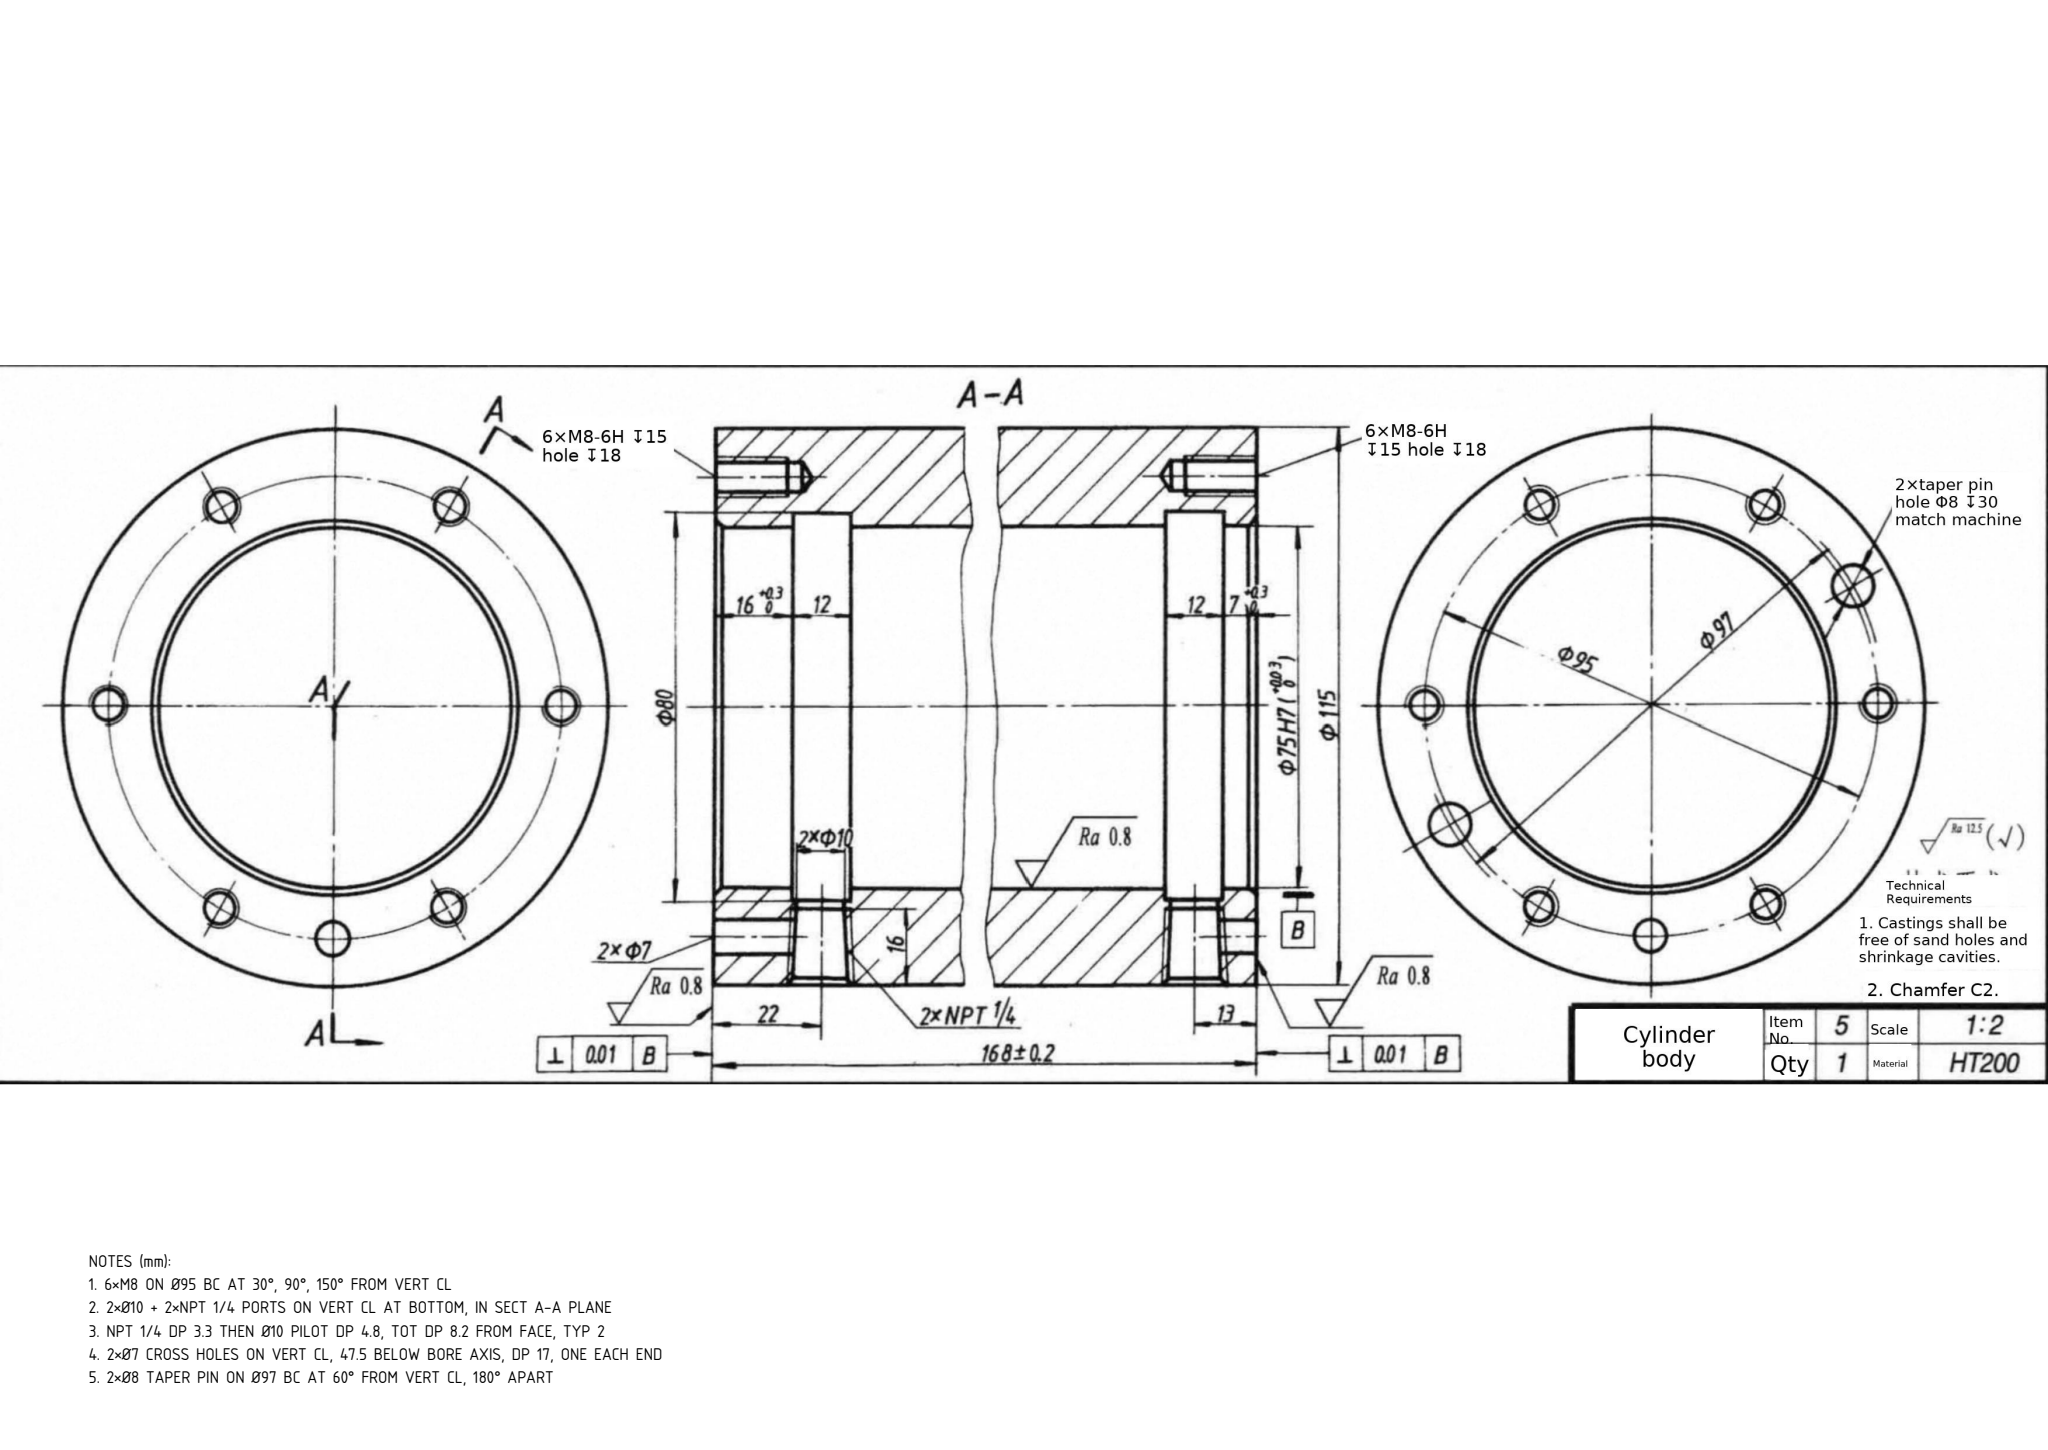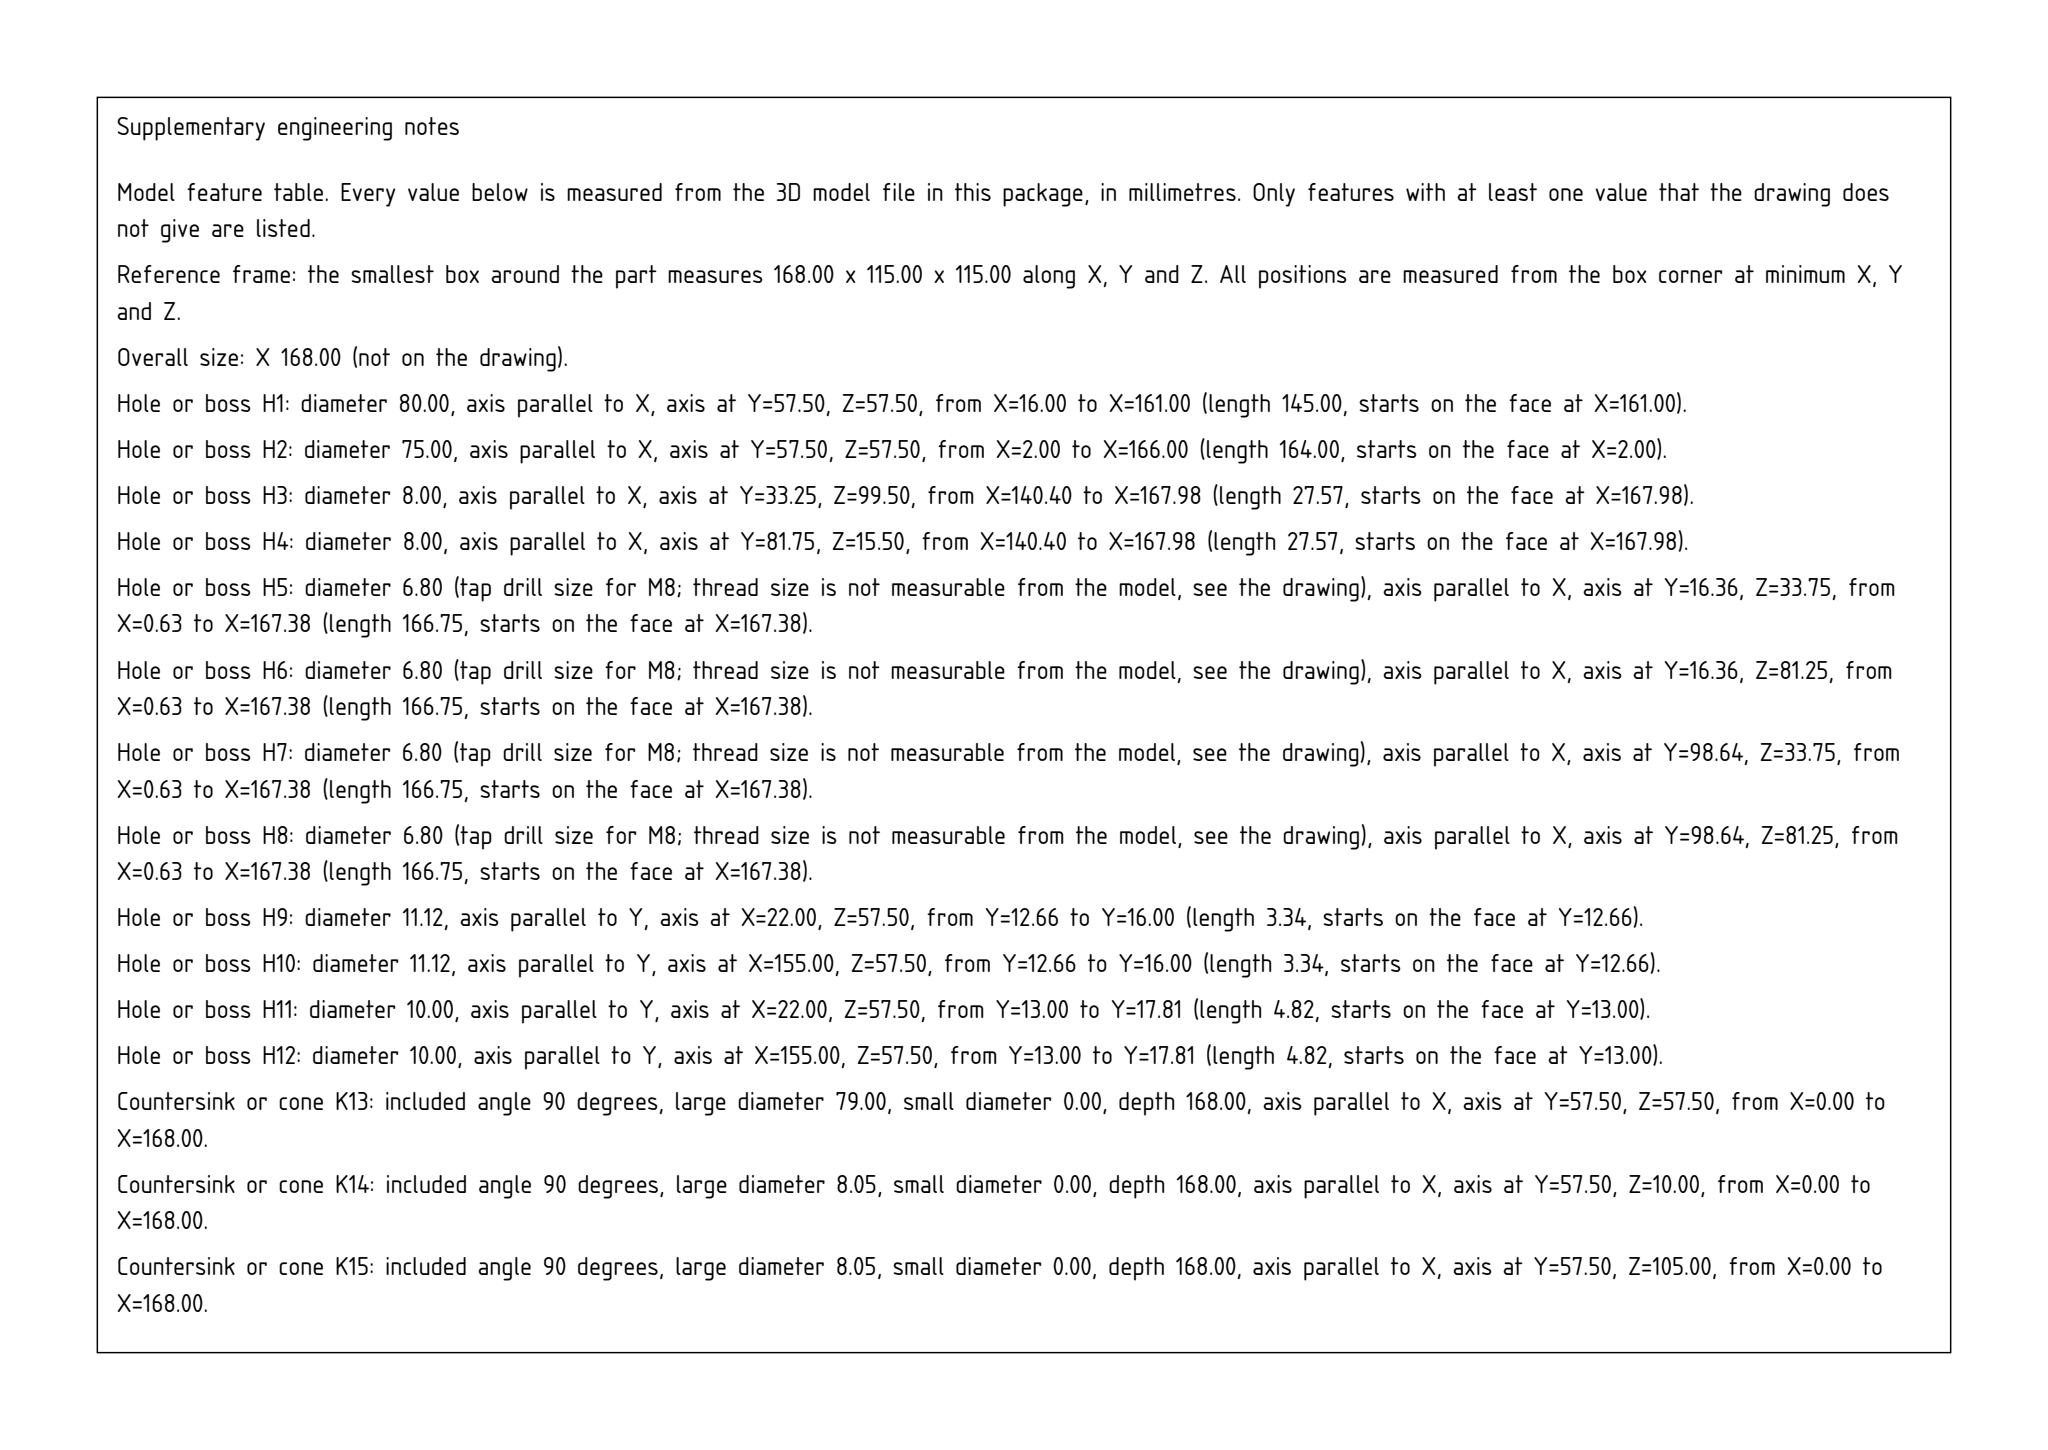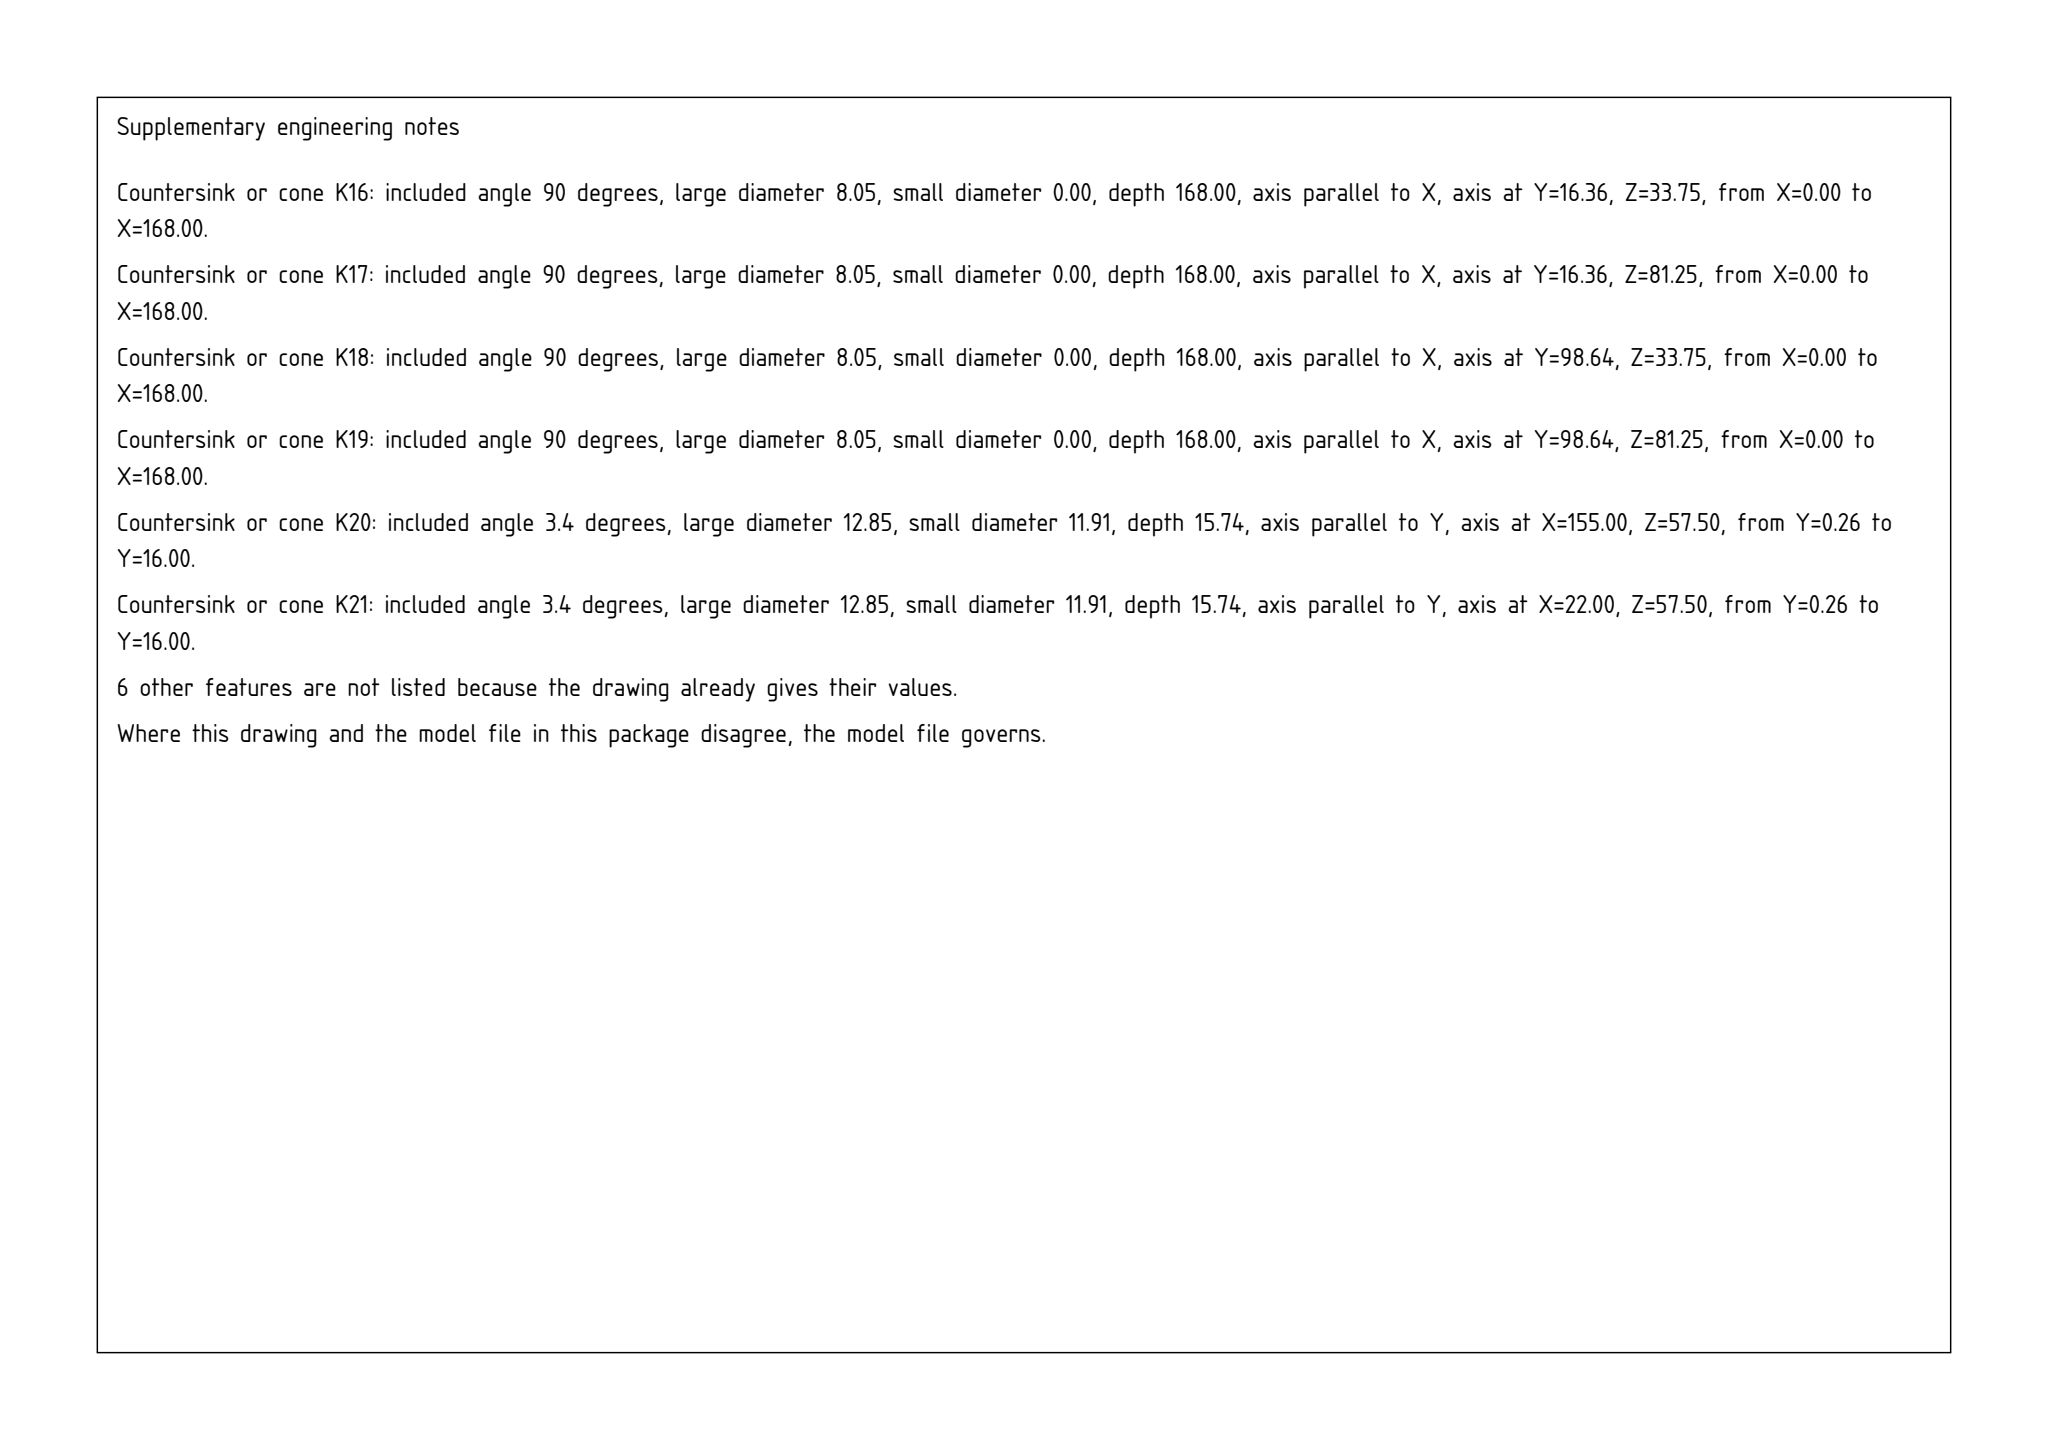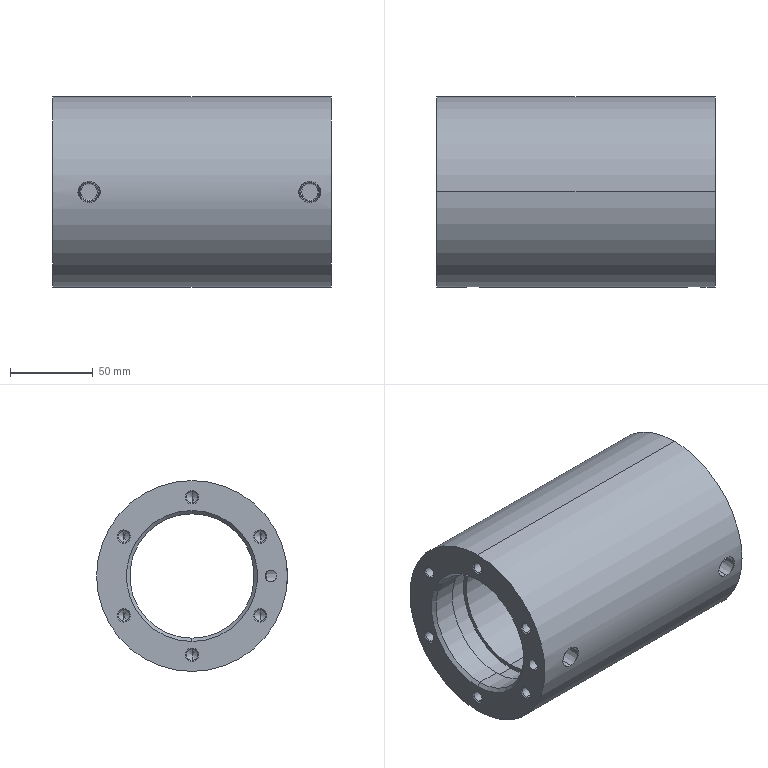Part | SolidWorks | mm | 1 solid | 136 faces | box 168 x 115 x 115 mm | volume 972210 mm3 | cone 74 | cylinder 54 | plane 8 | commonest cylinder face diameters 6.8 x24 7 x6 75 x6 10 x4 11.125 x4 8 x4 80 x4 115 x2
Drawing notes:
6×M8 ON Ø95 BC AT 30°, 90°, 150° FROM VERT CL | from the solid: 6×Ø6.8 tap drills at (16.36,33.75)(16.36,81.25)(57.5,10)(57.5,105)(98.64,33.75)(98.64,81.25), R47.5 from (57.5,57.5) => Ø95, 60° spacing
2×Ø10 + 2×NPT 1/4 PORTS ON VERT CL AT BOTTOM, IN SECT A-A PLANE | from the solid: Ø10/Ø11.125 cyls axis Y at x=22 & x=155, z=57.5; bore axis y=57.5,z=57.5 => radial, bottom side, 22 and 168-155=13 from ends
NPT 1/4 DP 3.3 THEN Ø10 PILOT DP 4.8, TOT DP 8.2 FROM FACE, TYP 2 | from the solid: Ø11.125 cyl axis y len 3.34 + Ø10 cyl axis y len 4.82 at x=22 and x=155, z=57.5; sum 8.16
2×Ø7 CROSS HOLES ON VERT CL, 47.5 BELOW BORE AXIS, DP 17, ONE EACH END | from the solid: Ø7 cyls axis X at y=10, z=57.5, len 16.97≈17 from end faces x=0 / x=168; 57.5-10=47.5 below bore axis
2×Ø8 TAPER PIN ON Ø97 BC AT 60° FROM VERT CL, 180° APART | from the solid: Ø8 holes at (33.25,99.5) & (81.75,15.5), R48.5 from (57.5,57.5) => Ø97, diametrically opposed
build123d program:
from build123d import *

# Parameters (mm, degrees)
M8_TAPPED_HOLE1_AT_2_COUNT         = 2
M8_TAPPED_HOLE1_AT_2_PITCH         = 47.5
M8_TAPPED_HOLE1_AT_3_COUNT         = 2
M8_TAPPED_HOLE1_AT_3_PITCH         = 82.272
M8_TAPPED_HOLE1_AT_4_COUNT         = 2
M8_TAPPED_HOLE1_AT_4_PITCH         = 95
M8_TAPPED_HOLE1_AT_5_COUNT         = 2
M8_TAPPED_HOLE1_AT_5_PITCH         = 82.272
M8_TAPPED_HOLE1_AT_6_COUNT         = 2
M8_TAPPED_HOLE1_AT_6_PITCH         = 47.5
HOLE1_D                            = 7
HOLE1_DEPTH                        = 22
HOLE2_D                            = 7
HOLE2_DEPTH                        = 13
CHAMFER1_SIZE                      = 2
F_8_0MM_DOWEL_HOLE1_D              = 8
F_8_0MM_DOWEL_HOLE1_DEPTH          = 27.597
F_8_0MM_DOWEL_HOLE1_CSINK_D        = 8.05
F_8_0MM_DOWEL_HOLE1_CSINK_ANGLE    = 90
F_8_0MM_DOWEL_HOLE1_TIP            = 2.403
F_1_4_NPT_TAPPED_HOLE15_AT_2_COUNT = 2
F_1_4_NPT_TAPPED_HOLE15_AT_2_PITCH = 133
SKETCH20_W                         = 5
SKETCH20_H                         = 35.696
SKETCH21_W                         = 5
SKETCH21_H                         = 37.567


with BuildPart() as part:
    # Sketch1 → Revolve1 (revolve)
    with BuildSketch(Plane.XY, mode=Mode.PRIVATE) as revolve1_sk:
        Polygon((0, 57.5), (0, 37.5), (16, 37.5), (16, 37.685), (16, 40), (28, 40), (28, 37.5), (149, 37.5), (149, 40), (161, 40), (161, 37.5), (168, 37.5), (168, 57.5), align=None)
    revolve(revolve1_sk.sketch.rotate(Axis((0, 0, 0), (1, 0, 0)), 90), axis=Axis((0, 0, 0), (1, 0, 0)))

    # Sketch3 → M8 Tapped Hole1 (revolve, cut)
    with BuildSketch(Plane(origin=(0, 41.136, -23.75), x_dir=(0, 0, 1), z_dir=(0, 1, 0))):
        Polygon((0, 0), (0, 18), (3.4, 15.957), (3.4, 0.625), (4.025, 0), align=None)
    m8_tapped_hole1 = revolve(axis=Axis((-6.35, 41.136, -23.75), (1, 0, 0)), mode=Mode.SUBTRACT)

    # M8 Tapped Hole1 at 2: M8 Tapped Hole1 ×2
    with Locations(*[Vector(0, -0.866, -0.5) * (i * M8_TAPPED_HOLE1_AT_2_PITCH) for i in range(1, M8_TAPPED_HOLE1_AT_2_COUNT)]):
        add(m8_tapped_hole1, mode=Mode.SUBTRACT)

    # M8 Tapped Hole1 at 3: M8 Tapped Hole1 ×2
    with Locations(*[(0, -i * M8_TAPPED_HOLE1_AT_3_PITCH, 0) for i in range(1, M8_TAPPED_HOLE1_AT_3_COUNT)]):
        add(m8_tapped_hole1, mode=Mode.SUBTRACT)

    # M8 Tapped Hole1 at 4: M8 Tapped Hole1 ×2
    with Locations(*[Vector(0, -0.866, 0.5) * (i * M8_TAPPED_HOLE1_AT_4_PITCH) for i in range(1, M8_TAPPED_HOLE1_AT_4_COUNT)]):
        add(m8_tapped_hole1, mode=Mode.SUBTRACT)

    # M8 Tapped Hole1 at 5: M8 Tapped Hole1 ×2
    with Locations(*[Vector(0, -0.5, 0.866) * (i * M8_TAPPED_HOLE1_AT_5_PITCH) for i in range(1, M8_TAPPED_HOLE1_AT_5_COUNT)]):
        add(m8_tapped_hole1, mode=Mode.SUBTRACT)

    # M8 Tapped Hole1 at 6: M8 Tapped Hole1 ×2
    with Locations(*[(0, 0, i * M8_TAPPED_HOLE1_AT_6_PITCH) for i in range(1, M8_TAPPED_HOLE1_AT_6_COUNT)]):
        add(m8_tapped_hole1, mode=Mode.SUBTRACT)

    # Hole1
    with Locations(Plane(origin=(0, -47.5, 0), x_dir=(0, 0, -1), z_dir=(-1, 0, 0))):
        with Locations((0, 0)):
            Hole(HOLE1_D / 2, depth=HOLE1_DEPTH)

    # Mirror1: M8 Tapped Hole1 across plane
    add(m8_tapped_hole1.mirror(Plane.ZY.offset(-84)), mode=Mode.SUBTRACT)

    # Mirror1 copy 1 sketch → Mirror1 copy 1 (revolve, cut)
    with BuildSketch(Plane(origin=(168, 0, -47.5), x_dir=(0, 0, 1), z_dir=(0, 1, 0))):
        Polygon((0, 0), (0, -18), (3.4, -15.957), (3.4, -0.625), (4.025, 0), align=None)
    revolve(axis=Axis((174.35, 0, -47.5), (1, 0, 0)), mode=Mode.SUBTRACT)

    # Mirror1 copy 2 sketch → Mirror1 copy 2 (revolve, cut)
    with BuildSketch(Plane(origin=(168, -41.136, -23.75), x_dir=(0, 0, 1), z_dir=(0, 1, 0))):
        Polygon((0, 0), (0, -18), (3.4, -15.957), (3.4, -0.625), (4.025, 0), align=None)
    revolve(axis=Axis((174.35, -41.136, -23.75), (1, 0, 0)), mode=Mode.SUBTRACT)

    # Mirror1 copy 3 sketch → Mirror1 copy 3 (revolve, cut)
    with BuildSketch(Plane(origin=(168, -41.136, 23.75), x_dir=(0, 0, 1), z_dir=(0, 1, 0))):
        Polygon((0, 0), (0, -18), (3.4, -15.957), (3.4, -0.625), (4.025, 0), align=None)
    revolve(axis=Axis((174.35, -41.136, 23.75), (1, 0, 0)), mode=Mode.SUBTRACT)

    # Mirror1 copy 4 sketch → Mirror1 copy 4 (revolve, cut)
    with BuildSketch(Plane(origin=(168, 0, 47.5), x_dir=(0, 0, 1), z_dir=(0, 1, 0))):
        Polygon((0, 0), (0, -18), (3.4, -15.957), (3.4, -0.625), (4.025, 0), align=None)
    revolve(axis=Axis((174.35, 0, 47.5), (1, 0, 0)), mode=Mode.SUBTRACT)

    # Mirror1 copy 5 sketch → Mirror1 copy 5 (revolve, cut)
    with BuildSketch(Plane(origin=(168, 41.136, 23.75), x_dir=(0, 0, 1), z_dir=(0, 1, 0))):
        Polygon((0, 0), (0, -18), (3.4, -15.957), (3.4, -0.625), (4.025, 0), align=None)
    revolve(axis=Axis((174.35, 41.136, 23.75), (1, 0, 0)), mode=Mode.SUBTRACT)

    # Hole2
    with Locations(Plane(origin=(168, 0, 0), x_dir=(0, 0, -1), z_dir=(1, 0, 0))):
        with Locations((0, -47.5)):
            Hole(HOLE2_D / 2, depth=HOLE2_DEPTH)

    # Chamfer1
    chamfer1_edges = [part.edges().sort_by_distance(p)[0] for p in [
        (0, 0, -37.5),
        (168, 0, -37.5),
    ]]
    chamfer(chamfer1_edges, length=CHAMFER1_SIZE)

    # 8.0mm Dowel Hole1
    with Locations(Plane(origin=(168, 0, 0), x_dir=(0, 0, -1), z_dir=(1, 0, 0))):
        with Locations((-42.002, -24.25), (42.002, 24.25)):
            CounterSinkHole(F_8_0MM_DOWEL_HOLE1_D / 2, F_8_0MM_DOWEL_HOLE1_CSINK_D / 2, depth=F_8_0MM_DOWEL_HOLE1_DEPTH, counter_sink_angle=F_8_0MM_DOWEL_HOLE1_CSINK_ANGLE)
            with Locations((0, 0, -(F_8_0MM_DOWEL_HOLE1_DEPTH + F_8_0MM_DOWEL_HOLE1_TIP / 2))):  # 118° drill point
                Cone(0, F_8_0MM_DOWEL_HOLE1_D / 2, F_8_0MM_DOWEL_HOLE1_TIP, mode=Mode.SUBTRACT)

    # Sketch17 → 1_4 NPT Tapped Hole15 (revolve, cut)
    with BuildSketch(Plane(origin=(22, -57.5, 0), x_dir=(0, 0, -1), z_dir=(1, 0, 0))):
        Polygon((0, 0), (0, 16), (5.563, 12.658), (5.563, 16), (5.951, 16), (6.423, 0.2587), (6.731, 0), align=None)
    f_1_4_npt_tapped_hole15 = revolve(axis=Axis((22, -63.85, 0), (0, 1, 0)), mode=Mode.SUBTRACT)

    # 1_4 NPT Tapped Hole15 at 2: 1_4 NPT Tapped Hole15 ×2
    with Locations(*[(i * F_1_4_NPT_TAPPED_HOLE15_AT_2_PITCH, 0, 0) for i in range(1, F_1_4_NPT_TAPPED_HOLE15_AT_2_COUNT)]):
        add(f_1_4_npt_tapped_hole15, mode=Mode.SUBTRACT)

    # Sketch20 → Cut-Revolve4 (revolve, cut)
    with BuildSketch(Plane(origin=(155, 0, 0), x_dir=(0, 0, -1), z_dir=(1, 0, 0))):
        with Locations((-2.5, -48.483)):
            Rectangle(SKETCH20_W, SKETCH20_H)
    revolve(axis=Axis((155, 0, 0), (0, -1, 0)), mode=Mode.SUBTRACT)

    # Sketch21 → Cut-Revolve5 (revolve, cut)
    with BuildSketch(Plane.ZY.offset(-22), mode=Mode.PRIVATE) as cut_revolve5_sk:
        with Locations((-2.5, -52.246)):
            Rectangle(SKETCH21_W, SKETCH21_H)
    revolve(cut_revolve5_sk.sketch.rotate(Axis((22, 0, 0), (0, -1, 0)), 180), axis=Axis((22, 0, 0), (0, -1, 0)), mode=Mode.SUBTRACT)


solid = part.part